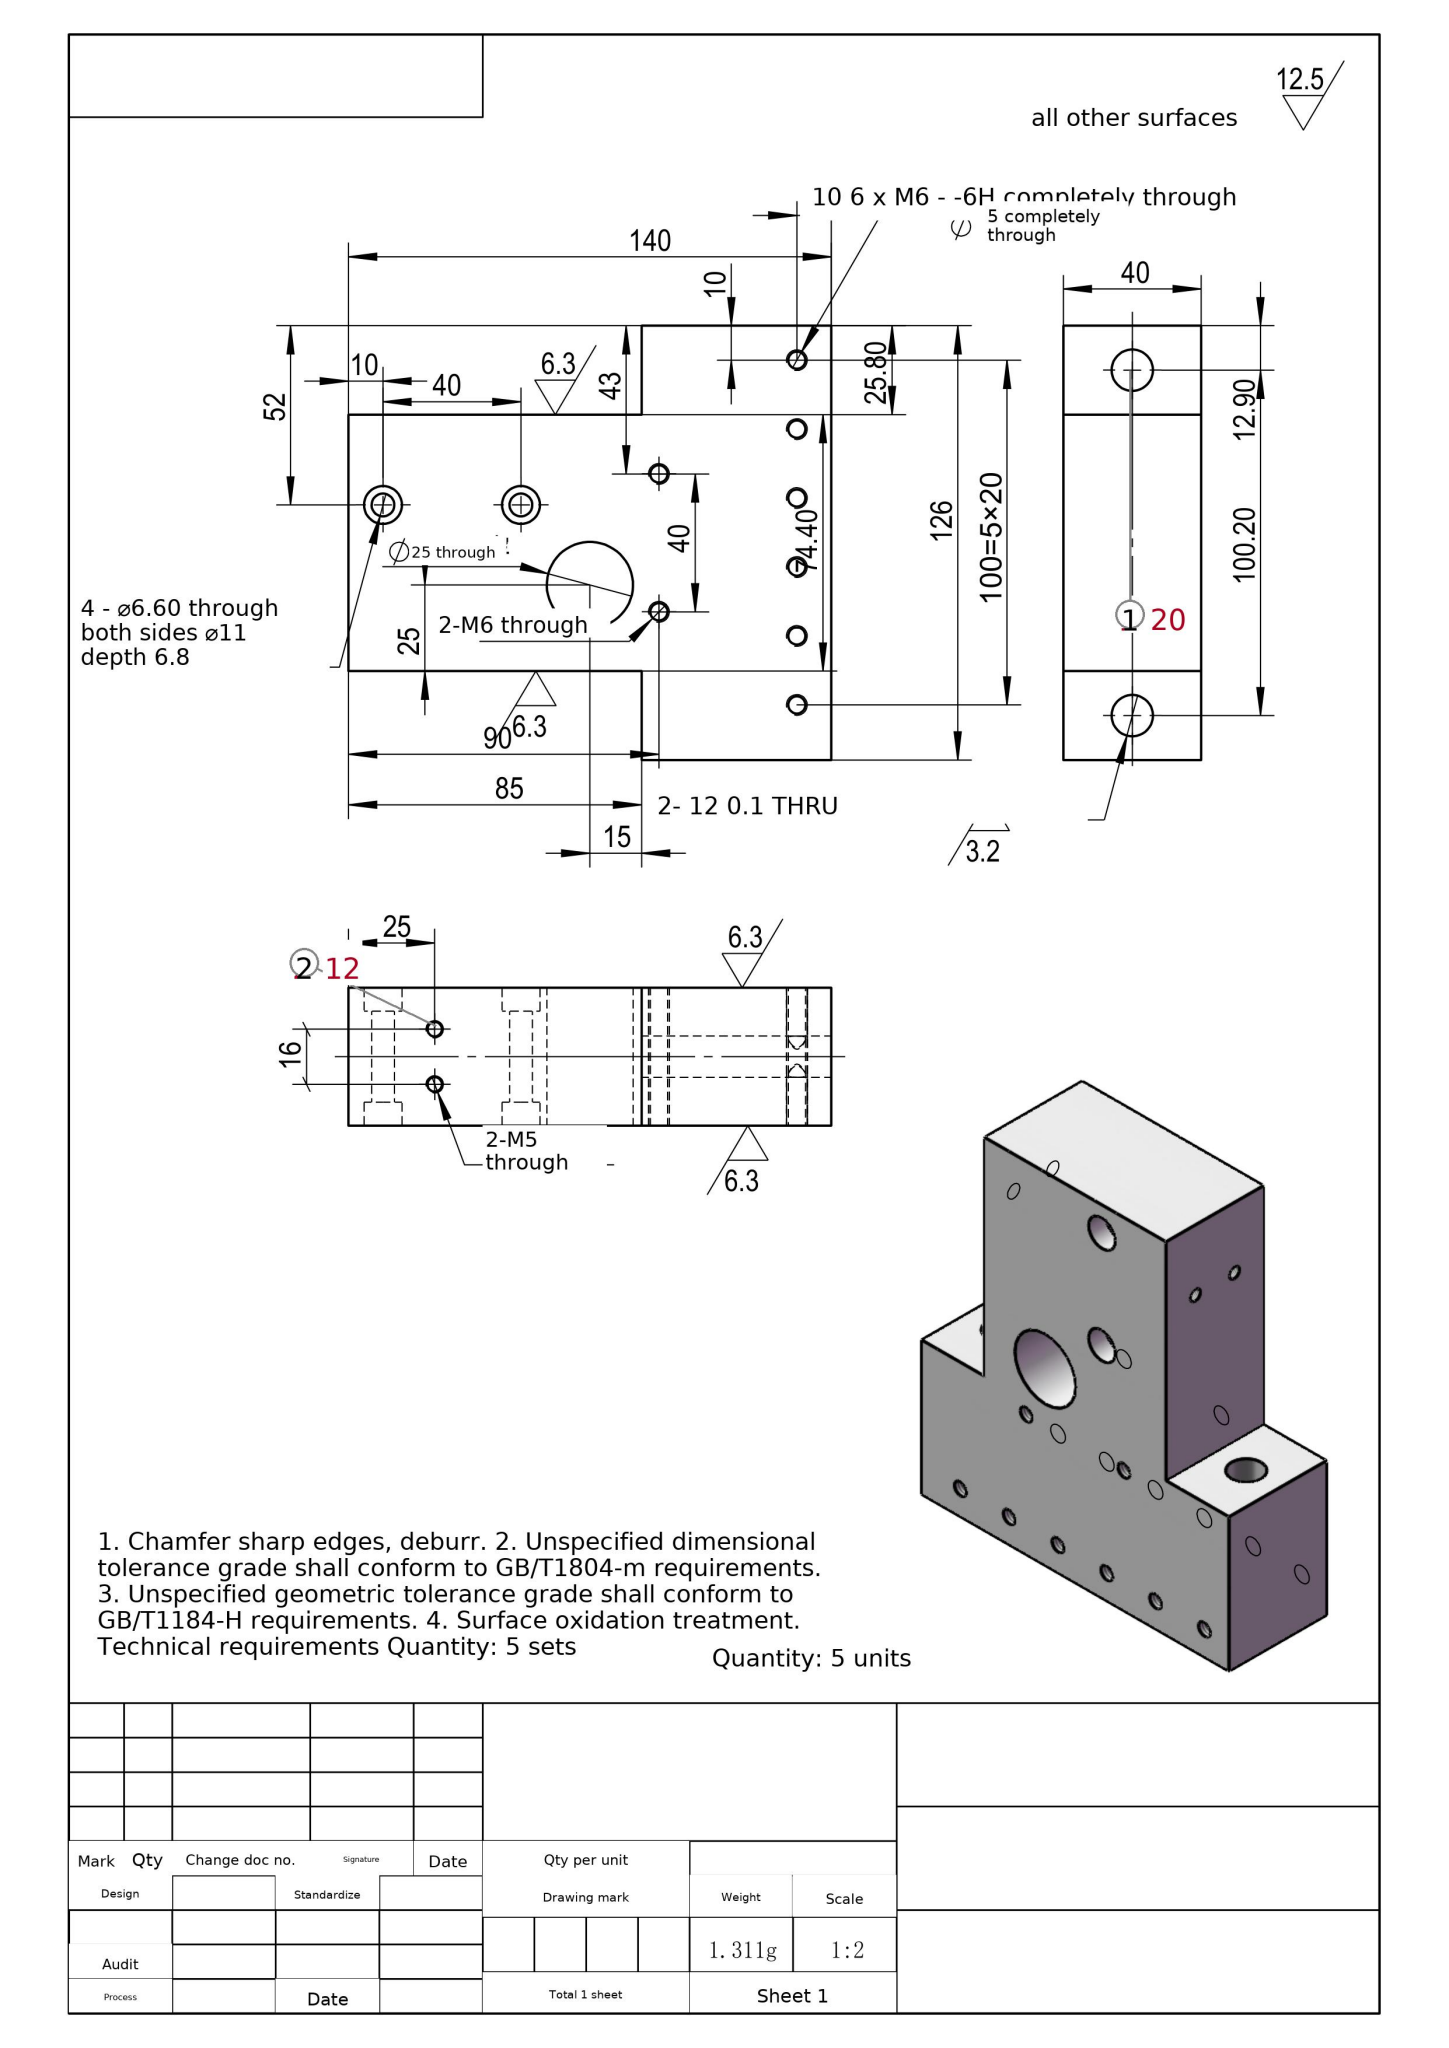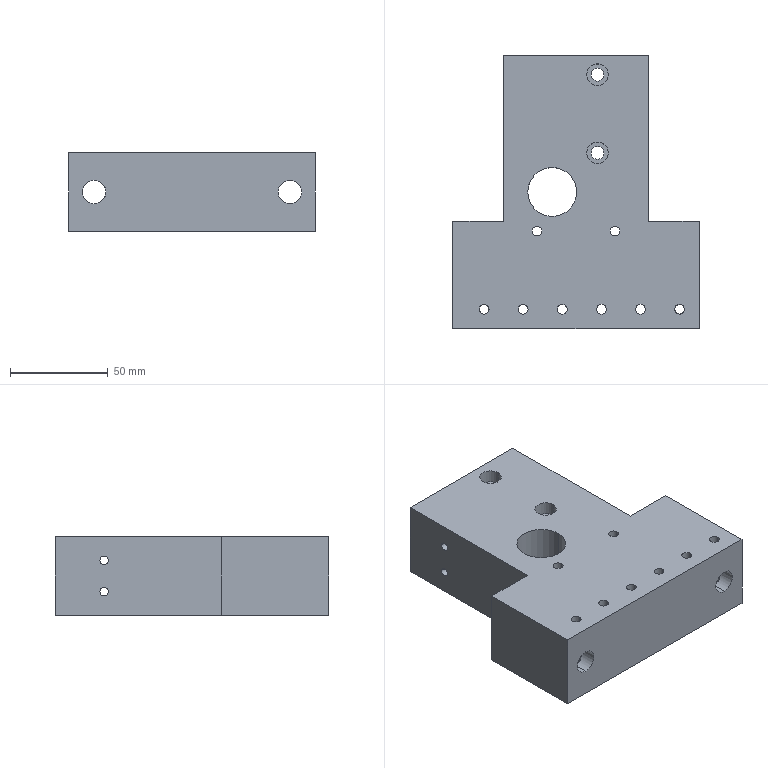Part | SolidWorks | mm | 1 solid | 56 faces | box 126 x 140 x 40 mm | volume 485739 mm3 | cylinder 42 | plane 14 | commonest cylinder face diameters 5 x20 11 x8 6.6 x4 12 x4 4.2 x4 25 x2
build123d program:
from build123d import *

# Parameters (mm, degrees)
SKETCH1_W                                           = 126
SKETCH1_H                                           = 140
BOSS_EXTRUDE1_DEPTH                                 = 20
SKETCH8_R                                           = 3
CUT_EXTRUDE1_DEPTH                                  = 103.318
SKETCH9_W                                           = 25.8
SKETCH9_H                                           = 85
CUT_EXTRUDE2_DEPTH                                  = 103.318
SKETCH10_R                                          = 4.5
CUT_EXTRUDE3_DEPTH                                  = 108.675
SKETCH11_R                                          = 2.1
CUT_EXTRUDE4_DEPTH                                  = 124.855
SKETCH12_R                                          = 6
CUT_EXTRUDE5_DEPTH                                  = 155.819
HOLE_SIZE_ACCORDING_TO_TYPE_1_OF_HEXAGO_D           = 6.6
HOLE_SIZE_ACCORDING_TO_TYPE_1_OF_HEXAGO_CBORE_D     = 11
HOLE_SIZE_ACCORDING_TO_TYPE_1_OF_HEXAGO_CBORE_DEPTH = 6.8
M6_TAPPED_HOLE1_D                                   = 5
M6_TAPPED_HOLE2_D                                   = 5
SKETCH21_R                                          = 12.5
CUT_EXTRUDE6_DEPTH                                  = 103.318


with BuildPart() as part:
    # Sketch1 → Boss-Extrude1 (new, symmetric)
    with BuildSketch(Plane.XY):
        Rectangle(SKETCH1_W, SKETCH1_H)
    extrude(amount=BOSS_EXTRUDE1_DEPTH, both=True)

    # Sketch8 → Cut-Extrude1 (cut, through all)
    with BuildSketch(Plane.XY.offset(20)):
        with Locations((11, 60)):
            Circle(SKETCH8_R)
        with Locations((11, 20)):
            Circle(SKETCH8_R)
    extrude(amount=-CUT_EXTRUDE1_DEPTH, mode=Mode.SUBTRACT)

    # Sketch9 → Cut-Extrude2 (cut, through all)
    with BuildSketch(Plane.XY.offset(20)):
        with Locations((50.1, 27.5)):
            Rectangle(SKETCH9_W, SKETCH9_H)
    cut_extrude2 = extrude(amount=-CUT_EXTRUDE2_DEPTH, mode=Mode.SUBTRACT)

    # Mirror1: Cut-Extrude2 across plane
    add(cut_extrude2.mirror(Plane(origin=(0, 0, 0), x_dir=(0, 0, 1), z_dir=(1, 0, 0))), mode=Mode.SUBTRACT)

    # Sketch10 → Cut-Extrude3 (cut, through all)
    with BuildSketch(Plane(origin=(0, -15, 0), x_dir=(-1, 0, 0), z_dir=(0, 1, 0))):
        with Locations((50.1, 0)):
            Circle(SKETCH10_R)
    cut_extrude3 = extrude(amount=-CUT_EXTRUDE3_DEPTH, mode=Mode.SUBTRACT)

    # Mirror2: Cut-Extrude3 across plane
    add(cut_extrude3.mirror(Plane(origin=(0, 0, 0), x_dir=(0, 0, 1), z_dir=(1, 0, 0))), mode=Mode.SUBTRACT)

    # Sketch11 → Cut-Extrude4 (cut, through all)
    with BuildSketch(Plane(origin=(37.2, 0, 0), x_dir=(0, 0, -1), z_dir=(1, 0, 0))):
        with Locations(Location((-8, 45, 0), (0, 0, 90))):
            Circle(SKETCH11_R)
        with Locations(Location((8, 45, 0), (0, 0, 90))):
            Circle(SKETCH11_R)
    extrude(amount=-CUT_EXTRUDE4_DEPTH, mode=Mode.SUBTRACT)

    # Sketch12 → Cut-Extrude5 (cut, through all)
    with BuildSketch(Plane.XZ.offset(70)):
        with Locations(Location((-50.1, 0, 0), (0, 0, 270))):
            Circle(SKETCH12_R)
    cut_extrude5 = extrude(amount=-CUT_EXTRUDE5_DEPTH, mode=Mode.SUBTRACT)

    # Mirror3: Cut-Extrude5 across plane
    add(cut_extrude5.mirror(Plane(origin=(0, 0, 0), x_dir=(0, 0, 1), z_dir=(1, 0, 0))), mode=Mode.SUBTRACT)

    # Hole Size_According to_ Type 1 of Hexago (through all)
    with Locations(Plane(origin=(0, 0, -20), x_dir=(-1, 0, 0), z_dir=(0, 0, -1))):
        with Locations((-11, 60), (-11, 20)):
            hole_size_according_to_type_1_of_hexago = CounterBoreHole(HOLE_SIZE_ACCORDING_TO_TYPE_1_OF_HEXAGO_D / 2, HOLE_SIZE_ACCORDING_TO_TYPE_1_OF_HEXAGO_CBORE_D / 2, HOLE_SIZE_ACCORDING_TO_TYPE_1_OF_HEXAGO_CBORE_DEPTH)

    # Mirror4: Hole Size_According to_ Type 1 of Hexago across plane
    add(hole_size_according_to_type_1_of_hexago.mirror(Plane.XY), mode=Mode.SUBTRACT)

    # M6 Tapped Hole1 (through all)
    with Locations(Plane(origin=(0, 0, -20), x_dir=(-1, 0, 0), z_dir=(0, 0, -1))):
        with Locations((-20, -20), (20, -20)):
            Hole(M6_TAPPED_HOLE1_D / 2)

    # M6 Tapped Hole2 (through all)
    with Locations(Plane(origin=(0, 0, -20), x_dir=(-1, 0, 0), z_dir=(0, 0, -1))):
        with Locations((-53, -60), (-33, -60), (-13, -60), (7, -60), (27, -60), (47, -60)):
            Hole(M6_TAPPED_HOLE2_D / 2)

    # Sketch21 → Cut-Extrude6 (cut, through all)
    with BuildSketch(Plane(origin=(0, 0, -20), x_dir=(-1, 0, 0), z_dir=(0, 0, -1))):
        with Locations((12.2, 0)):
            Circle(SKETCH21_R)
    extrude(amount=-CUT_EXTRUDE6_DEPTH, mode=Mode.SUBTRACT)


solid = part.part